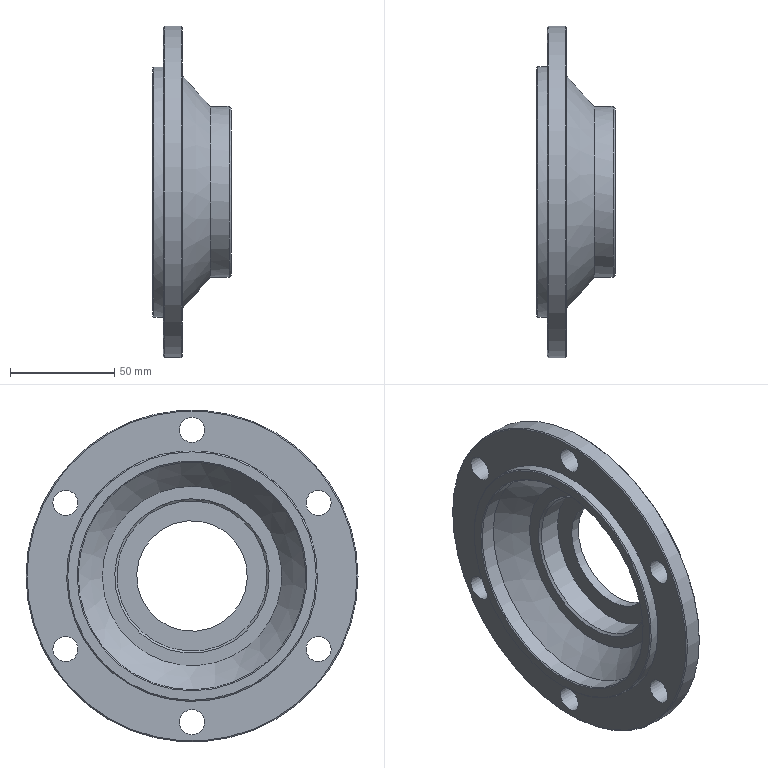Component | NX | FRONT_END_COVER | 1 solid | 26 faces | volume 151107 mm3 | cylinder 12 | cone 8 | plane 6 | commonest cylinder face diameters 12 x6 159 x1 120 x1 109 x1 53 x1 72 x1 82 x1